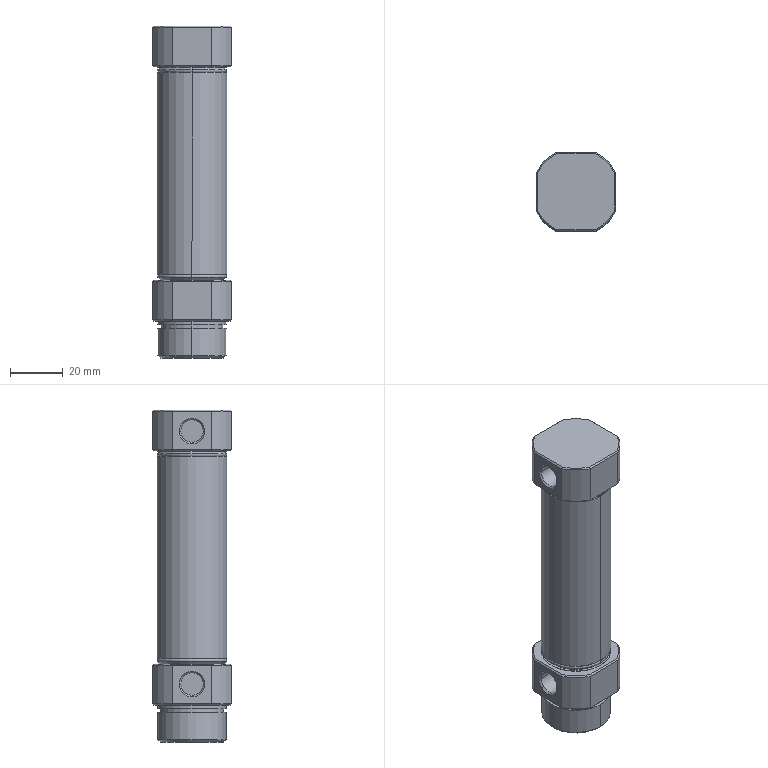Component | SolidWorks | MF_25x50_S_U_M_2_0-1_MF_25x50_S_U_c-1 | 1 solid | 99 faces | box 30 x 30 x 126 mm | volume 41442 mm3 | plane 37 | cone 30 | cylinder 28 | torus 4 | commonest cylinder face diameters 33.5 x8 26.4 x6 8.566 x4 26 x4 25 x2 10 x2 23.92 x2
build123d program:
from build123d import *

# Parameters (mm, degrees)
CUT_EXTRUDE1_START       = 15.5
SKETCH2_W                = 60
SKETCH2_H                = 60
CUT_EXTRUDE1_DEPTH       = 15.5
SKETCH3_W                = 60
SKETCH3_H                = 60
CUT_EXTRUDE2_DEPTH       = 15.5
CUT_EXTRUDE3_DEPTH       = 15
CUT_EXTRUDE3_DEPTH_BACK  = 15
CUT_EXTRUDE4_DEPTH       = 15
CUT_EXTRUDE4_DEPTH_BACK  = 15
CUT_EXTRUDE5_DEPTH       = 15
CUT_EXTRUDE5_DEPTH_BACK  = 15
CUT_EXTRUDE6_DEPTH       = 15
CUT_EXTRUDE6_DEPTH_BACK  = 15
CUT_EXTRUDE7_DEPTH       = 15
CUT_EXTRUDE7_DEPTH_BACK  = 15
CUT_EXTRUDE8_DEPTH       = 15
CUT_EXTRUDE8_DEPTH_BACK  = 15
CUT_EXTRUDE9_DEPTH       = 15
CUT_EXTRUDE9_DEPTH_BACK  = 15
CUT_EXTRUDE10_DEPTH      = 15
CUT_EXTRUDE10_DEPTH_BACK = 15
CUT_EXTRUDE11_DEPTH      = 15
CUT_EXTRUDE11_DEPTH_BACK = 15
CUT_EXTRUDE12_DEPTH      = 15
CUT_EXTRUDE12_DEPTH_BACK = 15
CUT_EXTRUDE13_DEPTH      = 15
CUT_EXTRUDE13_DEPTH_BACK = 15
CUT_EXTRUDE14_DEPTH      = 15
CUT_EXTRUDE14_DEPTH_BACK = 15
CUT_EXTRUDE15_DEPTH      = 15
CUT_EXTRUDE15_DEPTH_BACK = 15
CUT_EXTRUDE16_DEPTH      = 15
CUT_EXTRUDE16_DEPTH_BACK = 15
CUT_EXTRUDE17_DEPTH      = 15
CUT_EXTRUDE17_DEPTH_BACK = 15
CUT_EXTRUDE18_DEPTH      = 15
CUT_EXTRUDE18_DEPTH_BACK = 15


with BuildPart() as part:
    # Sketch1 → Revolve1 (revolve)
    with BuildSketch(Plane.XY, mode=Mode.PRIVATE) as revolve1_sk:
        with BuildLine():
            Line((0, 0), (0, 16.25))
            Line((0, 16.25), (0.5, 16.75))
            Line((0.5, 16.75), (15, 16.75))
            Line((15, 16.75), (15.5, 16.25))
            Line((15.5, 16.25), (15.5, 13.2))
            Line((15.5, 13.2), (15.6, 13.2))
            Line((15.6, 13.2), (15.6, 12.2))
            Line((15.6, 12.2), (16.5, 13))
            ThreePointArc((16.5, 13), (17.025, 13.198), (17.5, 12.9))
            Line((17.5, 12.9), (17.8, 13.2))
            Line((17.8, 13.2), (94.2, 13.2))
            Line((94.2, 13.2), (94.5, 12.9))
            ThreePointArc((94.5, 12.9), (94.975, 13.198), (95.5, 13))
            Line((95.5, 13), (96.4, 12.2))
            Line((96.4, 12.2), (96.4, 13.2))
            Line((96.4, 13.2), (96.5, 13.2))
            Line((96.5, 13.2), (96.5, 16.25))
            Line((96.5, 16.25), (97, 16.75))
            Line((97, 16.75), (111.5, 16.75))
            Line((111.5, 16.75), (112, 16.25))
            Line((112, 16.25), (112, 0))
            Line((112, 0), (0, 0))
        make_face()
    revolve(revolve1_sk.sketch.rotate(Axis((112, 0, 0), (-1, 0, 0)), 270), axis=Axis((112, 0, 0), (-1, 0, 0)))

    # Sketch2 → Cut-Extrude1 (cut)
    with BuildSketch(Plane(origin=(0, 0, 0), x_dir=(0, 0, -1), z_dir=(1, 0, 0)).offset(CUT_EXTRUDE1_START)):
        Rectangle(SKETCH2_W, SKETCH2_H)
        with BuildLine():
            Line((-15, 7.454), (-15, -7.454))
            ThreePointArc((-15, -7.454), (-11.844, -11.844), (-7.454, -15))
            Line((-7.454, -15), (7.454, -15))
            ThreePointArc((7.454, -15), (11.844, -11.844), (15, -7.454))
            Line((15, -7.454), (15, 7.454))
            ThreePointArc((15, 7.454), (11.844, 11.844), (7.454, 15))
            Line((7.454, 15), (-7.454, 15))
            ThreePointArc((-7.454, 15), (-11.844, 11.844), (-15, 7.454))
        make_face(mode=Mode.SUBTRACT)
    extrude(amount=-CUT_EXTRUDE1_DEPTH, mode=Mode.SUBTRACT)

    # Sketch3 → Cut-Extrude2 (cut)
    with BuildSketch(Plane(origin=(112, 0, 0), x_dir=(0, 0, -1), z_dir=(1, 0, 0))):
        Rectangle(SKETCH3_W, SKETCH3_H)
        with BuildLine():
            Line((-15, 7.454), (-15, -7.454))
            ThreePointArc((-15, -7.454), (-11.844, -11.844), (-7.454, -15))
            Line((-7.454, -15), (7.454, -15))
            ThreePointArc((7.454, -15), (11.844, -11.844), (15, -7.454))
            Line((15, -7.454), (15, 7.454))
            ThreePointArc((15, 7.454), (11.844, 11.844), (7.454, 15))
            Line((7.454, 15), (-7.454, 15))
            ThreePointArc((-7.454, 15), (-11.844, 11.844), (-15, 7.454))
        make_face(mode=Mode.SUBTRACT)
    extrude(amount=-CUT_EXTRUDE2_DEPTH, mode=Mode.SUBTRACT)

    # Sketch4 → Revolve2 (revolve)
    with BuildSketch(Plane.XY, mode=Mode.PRIVATE) as revolve2_sk:
        Polygon((-14, 0), (-14, 12.08), (-13.08, 13), (-2.8, 13), (-2.8, 11.96), (-1.4, 11.96), (-1.4, 13), (0, 13), (0, 0), align=None)
    revolve(revolve2_sk.sketch.rotate(Axis((0, 0, 0), (-1, 0, 0)), 270), axis=Axis((0, 0, 0), (-1, 0, 0)))

    # Sketch5 → Cut-Revolve1 (revolve, cut)
    with BuildSketch(Plane.XY, mode=Mode.PRIVATE) as cut_revolve1_sk:
        Polygon((-19, 0), (-19, 5), (24.4, 5), (24.4, 12.5), (88, 12.5), (88, 0), align=None)
    revolve(cut_revolve1_sk.sketch.rotate(Axis((88, 0, 0), (-1, 0, 0)), 270), axis=Axis((88, 0, 0), (-1, 0, 0)), mode=Mode.SUBTRACT)

    # Sketch6 → Cut-Revolve2 (revolve, cut)
    with BuildSketch(Plane.XY, mode=Mode.PRIVATE) as cut_revolve2_sk:
        Polygon((8, 7), (3.717, 7), (3.717, 14.419), (3.136, 15), (8, 15), align=None)
    revolve(cut_revolve2_sk.sketch.rotate(Axis((8, 15, 0), (0, -1, 0)), 90), axis=Axis((8, 15, 0), (0, -1, 0)), mode=Mode.SUBTRACT)

    # Sketch7 → Cut-Revolve3 (revolve, cut)
    with BuildSketch(Plane.XY, mode=Mode.PRIVATE) as cut_revolve3_sk:
        Polygon((104, 7), (99.717, 7), (99.717, 14.419), (99.136, 15), (104, 15), align=None)
    revolve(cut_revolve3_sk.sketch.rotate(Axis((104, 15, 0), (0, -1, 0)), 90), axis=Axis((104, 15, 0), (0, -1, 0)), mode=Mode.SUBTRACT)

    # Sketch8 → Cut-Extrude3 (cut, two sides: drawn at the far end of the back side and taken through both)
    with BuildSketch(Plane.XY.offset(-CUT_EXTRUDE3_DEPTH_BACK)):
        Polygon((0, 14.5), (0.5, 15), (0, 15), align=None)
    extrude(amount=CUT_EXTRUDE3_DEPTH + CUT_EXTRUDE3_DEPTH_BACK, mode=Mode.SUBTRACT)

    # Sketch9 → Cut-Extrude4 (cut, two sides: drawn at the far end of the back side and taken through both)
    with BuildSketch(Plane.XY.offset(-CUT_EXTRUDE4_DEPTH_BACK)):
        Polygon((0, -14.5), (0, -15), (0.5, -15), align=None)
    extrude(amount=CUT_EXTRUDE4_DEPTH + CUT_EXTRUDE4_DEPTH_BACK, mode=Mode.SUBTRACT)

    # Sketch10 → Cut-Extrude5 (cut, two sides: drawn at the far end of the back side and taken through both)
    with BuildSketch(Plane(origin=(0, 0, 0), x_dir=(1, 0, 0), z_dir=(0, 1, 0)).offset(-CUT_EXTRUDE5_DEPTH_BACK)):
        Polygon((0, 14.5), (0.5, 15), (0, 15), align=None)
    extrude(amount=CUT_EXTRUDE5_DEPTH + CUT_EXTRUDE5_DEPTH_BACK, mode=Mode.SUBTRACT)

    # Sketch11 → Cut-Extrude6 (cut, two sides: drawn at the far end of the back side and taken through both)
    with BuildSketch(Plane(origin=(0, 0, 0), x_dir=(1, 0, 0), z_dir=(0, 1, 0)).offset(-CUT_EXTRUDE6_DEPTH_BACK)):
        Polygon((0, -14.5), (0, -15), (0.5, -15), align=None)
    extrude(amount=CUT_EXTRUDE6_DEPTH + CUT_EXTRUDE6_DEPTH_BACK, mode=Mode.SUBTRACT)

    # Sketch12 → Cut-Extrude7 (cut, two sides: drawn at the far end of the back side and taken through both)
    with BuildSketch(Plane.XY.offset(-CUT_EXTRUDE7_DEPTH_BACK)):
        Polygon((15, 15), (15.5, 14.5), (15.5, 15), align=None)
    extrude(amount=CUT_EXTRUDE7_DEPTH + CUT_EXTRUDE7_DEPTH_BACK, mode=Mode.SUBTRACT)

    # Sketch13 → Cut-Extrude8 (cut, two sides: drawn at the far end of the back side and taken through both)
    with BuildSketch(Plane.XY.offset(-CUT_EXTRUDE8_DEPTH_BACK)):
        Polygon((15, -15), (15.5, -15), (15.5, -14.5), align=None)
    extrude(amount=CUT_EXTRUDE8_DEPTH + CUT_EXTRUDE8_DEPTH_BACK, mode=Mode.SUBTRACT)

    # Sketch14 → Cut-Extrude9 (cut, two sides: drawn at the far end of the back side and taken through both)
    with BuildSketch(Plane(origin=(0, 0, 0), x_dir=(1, 0, 0), z_dir=(0, 1, 0)).offset(-CUT_EXTRUDE9_DEPTH_BACK)):
        Polygon((15, 15), (15.5, 14.5), (15.5, 15), align=None)
    extrude(amount=CUT_EXTRUDE9_DEPTH + CUT_EXTRUDE9_DEPTH_BACK, mode=Mode.SUBTRACT)

    # Sketch15 → Cut-Extrude10 (cut, two sides: drawn at the far end of the back side and taken through both)
    with BuildSketch(Plane(origin=(0, 0, 0), x_dir=(1, 0, 0), z_dir=(0, 1, 0)).offset(-CUT_EXTRUDE10_DEPTH_BACK)):
        Polygon((15, -15), (15.5, -15), (15.5, -14.5), align=None)
    extrude(amount=CUT_EXTRUDE10_DEPTH + CUT_EXTRUDE10_DEPTH_BACK, mode=Mode.SUBTRACT)

    # Sketch16 → Cut-Extrude11 (cut, two sides: drawn at the far end of the back side and taken through both)
    with BuildSketch(Plane.XY.offset(-CUT_EXTRUDE11_DEPTH_BACK)):
        Polygon((111.5, 15), (112, 14.5), (112, 15), align=None)
    extrude(amount=CUT_EXTRUDE11_DEPTH + CUT_EXTRUDE11_DEPTH_BACK, mode=Mode.SUBTRACT)

    # Sketch17 → Cut-Extrude12 (cut, two sides: drawn at the far end of the back side and taken through both)
    with BuildSketch(Plane.XY.offset(-CUT_EXTRUDE12_DEPTH_BACK)):
        Polygon((111.5, -15), (112, -15), (112, -14.5), align=None)
    extrude(amount=CUT_EXTRUDE12_DEPTH + CUT_EXTRUDE12_DEPTH_BACK, mode=Mode.SUBTRACT)

    # Sketch18 → Cut-Extrude13 (cut, two sides: drawn at the far end of the back side and taken through both)
    with BuildSketch(Plane(origin=(0, 0, 0), x_dir=(1, 0, 0), z_dir=(0, 1, 0)).offset(-CUT_EXTRUDE13_DEPTH_BACK)):
        Polygon((111.5, 15), (112, 14.5), (112, 15), align=None)
    extrude(amount=CUT_EXTRUDE13_DEPTH + CUT_EXTRUDE13_DEPTH_BACK, mode=Mode.SUBTRACT)

    # Sketch19 → Cut-Extrude14 (cut, two sides: drawn at the far end of the back side and taken through both)
    with BuildSketch(Plane(origin=(0, 0, 0), x_dir=(1, 0, 0), z_dir=(0, 1, 0)).offset(-CUT_EXTRUDE14_DEPTH_BACK)):
        Polygon((111.5, -15), (112, -15), (112, -14.5), align=None)
    extrude(amount=CUT_EXTRUDE14_DEPTH + CUT_EXTRUDE14_DEPTH_BACK, mode=Mode.SUBTRACT)

    # Sketch20 → Cut-Extrude15 (cut, two sides: drawn at the far end of the back side and taken through both)
    with BuildSketch(Plane.XY.offset(-CUT_EXTRUDE15_DEPTH_BACK)):
        Polygon((96.5, 14.5), (97, 15), (96.5, 15), align=None)
    extrude(amount=CUT_EXTRUDE15_DEPTH + CUT_EXTRUDE15_DEPTH_BACK, mode=Mode.SUBTRACT)

    # Sketch21 → Cut-Extrude16 (cut, two sides: drawn at the far end of the back side and taken through both)
    with BuildSketch(Plane.XY.offset(-CUT_EXTRUDE16_DEPTH_BACK)):
        Polygon((96.5, -14.5), (96.5, -15), (97, -15), align=None)
    extrude(amount=CUT_EXTRUDE16_DEPTH + CUT_EXTRUDE16_DEPTH_BACK, mode=Mode.SUBTRACT)

    # Sketch22 → Cut-Extrude17 (cut, two sides: drawn at the far end of the back side and taken through both)
    with BuildSketch(Plane(origin=(0, 0, 0), x_dir=(1, 0, 0), z_dir=(0, 1, 0)).offset(-CUT_EXTRUDE17_DEPTH_BACK)):
        Polygon((96.5, 14.5), (97, 15), (96.5, 15), align=None)
    extrude(amount=CUT_EXTRUDE17_DEPTH + CUT_EXTRUDE17_DEPTH_BACK, mode=Mode.SUBTRACT)

    # Sketch23 → Cut-Extrude18 (cut, two sides: drawn at the far end of the back side and taken through both)
    with BuildSketch(Plane(origin=(0, 0, 0), x_dir=(1, 0, 0), z_dir=(0, 1, 0)).offset(-CUT_EXTRUDE18_DEPTH_BACK)):
        Polygon((96.5, -14.5), (96.5, -15), (97, -15), align=None)
    extrude(amount=CUT_EXTRUDE18_DEPTH + CUT_EXTRUDE18_DEPTH_BACK, mode=Mode.SUBTRACT)


solid = part.part

# Placed as in the assembly
solid = solid.moved(Location((-102.5, -29.5, 213), (90, 0, 90)))